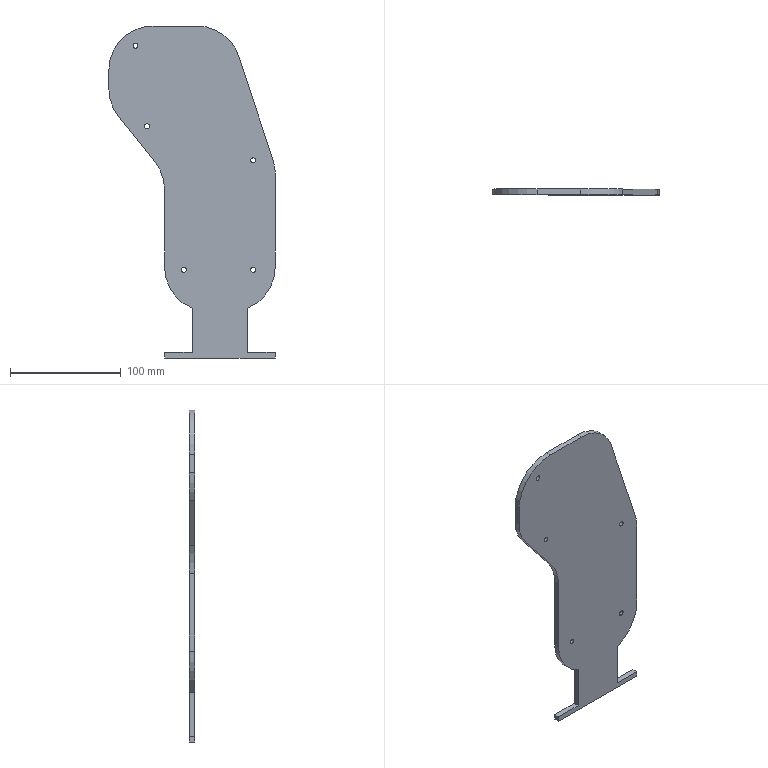Component | SolidWorks | FlatJawHousing-1 | 1 solid | 32 faces | box 150.39 x 5 x 300 mm | volume 146943 mm3 | cylinder 17 | plane 15 | commonest cylinder face diameters 4.5 x10 80 x7
build123d program:
from build123d import *

# Parameters (mm, degrees)
BOSS_EXTRUDE1_DEPTH = 5
SKETCH2_R           = 2.25
CUT_EXTRUDE1_DEPTH  = 10


with BuildPart() as part:
    # Sketch1 → Boss-Extrude1 (new body)
    with BuildSketch(Plane.XY):
        with BuildLine():
            Line((0, 111.584), (0, 95.56))
            Line((0, 95.56), (0, 52.34))
            Line((0, 52.34), (5, 52.34))
            Line((5, 52.34), (5, 77.34))
            Line((5, 77.34), (45, 77.34))
            ThreePointArc((45, 77.34), (59.72, 59.173), (82.081, 52.34))
            Line((82.081, 52.34), (152.399, 52.34))
            ThreePointArc((152.399, 52.34), (165.69, 50.067), (177.471, 43.507))
            Line((177.471, 43.507), (218.149, 10.784))
            ThreePointArc((218.149, 10.784), (229.929, 4.224), (243.221, 1.951))
            Line((243.221, 1.951), (260, 1.951))
            ThreePointArc((260, 1.951), (288.284, 13.667), (300, 41.951))
            Line((300, 41.951), (300, 81.523))
            ThreePointArc((300, 81.523), (292.396, 104.986), (272.474, 119.528))
            Line((272.474, 119.528), (178.577, 150.345))
            ThreePointArc((178.577, 150.345), (172.42, 151.838), (166.104, 152.34))
            Line((166.104, 152.34), (82.081, 152.34))
            ThreePointArc((82.081, 152.34), (59.72, 145.506), (45, 127.34))
            Line((45, 127.34), (5, 127.34))
            Line((5, 127.34), (5, 152.34))
            Line((5, 152.34), (0, 152.34))
            Line((0, 152.34), (0, 111.584))
        make_face()
    extrude(amount=BOSS_EXTRUDE1_DEPTH)

    # Sketch2 → Cut-Extrude1 (cut)
    with BuildSketch(Plane.XY.offset(5)):
        with Locations((79.643, 69.69)):
            Circle(SKETCH2_R)
        with Locations((79.643, 132.549)):
            Circle(SKETCH2_R)
        with Locations((178.581, 132.549)):
            Circle(SKETCH2_R)
        with Locations((209.296, 36.501)):
            Circle(SKETCH2_R)
        with Locations((282.295, 26.112)):
            Circle(SKETCH2_R)
    extrude(amount=-CUT_EXTRUDE1_DEPTH, mode=Mode.SUBTRACT)


solid = part.part

# Placed as in the assembly
solid = solid.moved(Location((361.097, 1552.5, -2182.934), (-90, 0, -90)))
STEP:
#1=COLOUR_RGB('',0.7922,0.8196,0.9333);
#2=FILL_AREA_STYLE_COLOUR('',#1);
#3=FILL_AREA_STYLE('',(#2));
#4=SURFACE_STYLE_FILL_AREA(#3);
#5=SURFACE_SIDE_STYLE('',(#4));
#6=SURFACE_STYLE_USAGE(.BOTH.,#5);
#7=PRESENTATION_STYLE_ASSIGNMENT((#6));
#8=CARTESIAN_POINT('',(15.244,61.122,-74.917));
#9=VERTEX_POINT('',#8);
#10=CARTESIAN_POINT('',(15.244,61.122,-74.74));
#11=VERTEX_POINT('',#10);
#12=CARTESIAN_POINT('',(15.244,61.122,-74.828));
#13=DIRECTION('',(0.,1.,-0.));
#14=DIRECTION('',(0.,0.,1.));
#15=AXIS2_PLACEMENT_3D('',#12,#13,#14);
#16=CIRCLE('',#15,0.08858);
#17=EDGE_CURVE('',#9,#11,#16,.T.);
#18=ORIENTED_EDGE('',*,*,#17,.F.);
#19=CARTESIAN_POINT('',(15.244,61.319,-74.917));
#20=VERTEX_POINT('',#19);
#21=CARTESIAN_POINT('',(15.244,60.925,-74.917));
#22=DIRECTION('',(0.,1.,-0.));
#23=VECTOR('',#22,39.37);
#24=LINE('',#21,#23);
#25=EDGE_CURVE('',#9,#20,#24,.T.);
#26=ORIENTED_EDGE('',*,*,#25,.T.);
#27=CARTESIAN_POINT('',(15.244,61.319,-74.74));
#28=VERTEX_POINT('',#27);
#29=CARTESIAN_POINT('',(15.244,61.319,-74.828));
#30=DIRECTION('',(0.,1.,-0.));
#31=DIRECTION('',(0.,0.,1.));
#32=AXIS2_PLACEMENT_3D('',#29,#30,#31);
#33=CIRCLE('',#32,0.08858);
#34=EDGE_CURVE('',#20,#28,#33,.T.);
#35=ORIENTED_EDGE('',*,*,#34,.T.);
#36=CARTESIAN_POINT('',(15.244,60.925,-74.74));
#37=DIRECTION('',(0.,1.,-0.));
#38=VECTOR('',#37,39.37);
#39=LINE('',#36,#38);
#40=EDGE_CURVE('',#11,#28,#39,.T.);
#41=ORIENTED_EDGE('',*,*,#40,.F.);
#42=EDGE_LOOP('',(#18,#26,#35,#41));
#43=FACE_OUTER_BOUND('',#42,.T.);
#44=CARTESIAN_POINT('',(15.244,60.925,-74.828));
#45=DIRECTION('',(0.,1.,-0.));
#46=DIRECTION('',(0.,0.,1.));
#47=AXIS2_PLACEMENT_3D('',#44,#45,#46);
#48=CYLINDRICAL_SURFACE('',#47,0.08858);
#49=ADVANCED_FACE('',(#43),#48,.F.);
#50=CARTESIAN_POINT('',(15.653,61.122,-77.791));
#51=VERTEX_POINT('',#50);
#52=CARTESIAN_POINT('',(15.653,61.122,-77.614));
#53=VERTEX_POINT('',#52);
#54=CARTESIAN_POINT('',(15.653,61.122,-77.702));
#55=DIRECTION('',(0.,1.,-0.));
#56=DIRECTION('',(0.,0.,1.));
#57=AXIS2_PLACEMENT_3D('',#54,#55,#56);
#58=CIRCLE('',#57,0.08858);
#59=EDGE_CURVE('',#51,#53,#58,.T.);
#60=ORIENTED_EDGE('',*,*,#59,.F.);
#61=CARTESIAN_POINT('',(15.653,61.319,-77.791));
#62=VERTEX_POINT('',#61);
#63=CARTESIAN_POINT('',(15.653,60.925,-77.791));
#64=DIRECTION('',(0.,1.,-0.));
#65=VECTOR('',#64,39.37);
#66=LINE('',#63,#65);
#67=EDGE_CURVE('',#51,#62,#66,.T.);
#68=ORIENTED_EDGE('',*,*,#67,.T.);
#69=CARTESIAN_POINT('',(15.653,61.319,-77.614));
#70=VERTEX_POINT('',#69);
#71=CARTESIAN_POINT('',(15.653,61.319,-77.702));
#72=DIRECTION('',(0.,1.,-0.));
#73=DIRECTION('',(0.,0.,1.));
#74=AXIS2_PLACEMENT_3D('',#71,#72,#73);
#75=CIRCLE('',#74,0.08858);
#76=EDGE_CURVE('',#62,#70,#75,.T.);
#77=ORIENTED_EDGE('',*,*,#76,.T.);
#78=CARTESIAN_POINT('',(15.653,60.925,-77.614));
#79=DIRECTION('',(0.,1.,-0.));
#80=VECTOR('',#79,39.37);
#81=LINE('',#78,#80);
#82=EDGE_CURVE('',#53,#70,#81,.T.);
#83=ORIENTED_EDGE('',*,*,#82,.F.);
#84=EDGE_LOOP('',(#60,#68,#77,#83));
#85=FACE_OUTER_BOUND('',#84,.T.);
#86=CARTESIAN_POINT('',(15.653,60.925,-77.702));
#87=DIRECTION('',(0.,1.,-0.));
#88=DIRECTION('',(0.,0.,1.));
#89=AXIS2_PLACEMENT_3D('',#86,#87,#88);
#90=CYLINDRICAL_SURFACE('',#89,0.08858);
#91=ADVANCED_FACE('',(#85),#90,.F.);
#92=CARTESIAN_POINT('',(19.435,61.122,-79.));
#93=VERTEX_POINT('',#92);
#94=CARTESIAN_POINT('',(19.435,61.122,-78.823));
#95=VERTEX_POINT('',#94);
#96=CARTESIAN_POINT('',(19.435,61.122,-78.912));
#97=DIRECTION('',(0.,1.,-0.));
#98=DIRECTION('',(0.,0.,1.));
#99=AXIS2_PLACEMENT_3D('',#96,#97,#98);
#100=CIRCLE('',#99,0.08858);
#101=EDGE_CURVE('',#93,#95,#100,.T.);
#102=ORIENTED_EDGE('',*,*,#101,.F.);
#103=CARTESIAN_POINT('',(19.435,61.319,-79.));
#104=VERTEX_POINT('',#103);
#105=CARTESIAN_POINT('',(19.435,60.925,-79.));
#106=DIRECTION('',(0.,1.,-0.));
#107=VECTOR('',#106,39.37);
#108=LINE('',#105,#107);
#109=EDGE_CURVE('',#93,#104,#108,.T.);
#110=ORIENTED_EDGE('',*,*,#109,.T.);
#111=CARTESIAN_POINT('',(19.435,61.319,-78.823));
#112=VERTEX_POINT('',#111);
#113=CARTESIAN_POINT('',(19.435,61.319,-78.912));
#114=DIRECTION('',(0.,1.,-0.));
#115=DIRECTION('',(0.,0.,1.));
#116=AXIS2_PLACEMENT_3D('',#113,#114,#115);
#117=CIRCLE('',#116,0.08858);
#118=EDGE_CURVE('',#104,#112,#117,.T.);
#119=ORIENTED_EDGE('',*,*,#118,.T.);
#120=CARTESIAN_POINT('',(19.435,60.925,-78.823));
#121=DIRECTION('',(0.,1.,-0.));
#122=VECTOR('',#121,39.37);
#123=LINE('',#120,#122);
#124=EDGE_CURVE('',#95,#112,#123,.T.);
#125=ORIENTED_EDGE('',*,*,#124,.F.);
#126=EDGE_LOOP('',(#102,#110,#119,#125));
#127=FACE_OUTER_BOUND('',#126,.T.);
#128=CARTESIAN_POINT('',(19.435,60.925,-78.912));
#129=DIRECTION('',(0.,1.,-0.));
#130=DIRECTION('',(0.,0.,1.));
#131=AXIS2_PLACEMENT_3D('',#128,#129,#130);
#132=CYLINDRICAL_SURFACE('',#131,0.08858);
#133=ADVANCED_FACE('',(#127),#132,.F.);
#134=CARTESIAN_POINT('',(19.435,61.122,-82.895));
#135=VERTEX_POINT('',#134);
#136=CARTESIAN_POINT('',(19.435,61.122,-82.718));
#137=VERTEX_POINT('',#136);
#138=CARTESIAN_POINT('',(19.435,61.122,-82.807));
#139=DIRECTION('',(0.,1.,-0.));
#140=DIRECTION('',(0.,0.,1.));
#141=AXIS2_PLACEMENT_3D('',#138,#139,#140);
#142=CIRCLE('',#141,0.08858);
#143=EDGE_CURVE('',#135,#137,#142,.T.);
#144=ORIENTED_EDGE('',*,*,#143,.F.);
#145=CARTESIAN_POINT('',(19.435,61.319,-82.895));
#146=VERTEX_POINT('',#145);
#147=CARTESIAN_POINT('',(19.435,60.925,-82.895));
#148=DIRECTION('',(0.,1.,-0.));
#149=VECTOR('',#148,39.37);
#150=LINE('',#147,#149);
#151=EDGE_CURVE('',#135,#146,#150,.T.);
#152=ORIENTED_EDGE('',*,*,#151,.T.);
#153=CARTESIAN_POINT('',(19.435,61.319,-82.718));
#154=VERTEX_POINT('',#153);
#155=CARTESIAN_POINT('',(19.435,61.319,-82.807));
#156=DIRECTION('',(0.,1.,-0.));
#157=DIRECTION('',(0.,0.,1.));
#158=AXIS2_PLACEMENT_3D('',#155,#156,#157);
#159=CIRCLE('',#158,0.08858);
#160=EDGE_CURVE('',#146,#154,#159,.T.);
#161=ORIENTED_EDGE('',*,*,#160,.T.);
#162=CARTESIAN_POINT('',(19.435,60.925,-82.718));
#163=DIRECTION('',(0.,1.,-0.));
#164=VECTOR('',#163,39.37);
#165=LINE('',#162,#164);
#166=EDGE_CURVE('',#137,#154,#165,.T.);
#167=ORIENTED_EDGE('',*,*,#166,.F.);
#168=EDGE_LOOP('',(#144,#152,#161,#167));
#169=FACE_OUTER_BOUND('',#168,.T.);
#170=CARTESIAN_POINT('',(19.435,60.925,-82.807));
#171=DIRECTION('',(0.,1.,-0.));
#172=DIRECTION('',(0.,0.,1.));
#173=AXIS2_PLACEMENT_3D('',#170,#171,#172);
#174=CYLINDRICAL_SURFACE('',#173,0.08858);
#175=ADVANCED_FACE('',(#169),#174,.F.);
#176=CARTESIAN_POINT('',(16.96,61.122,-82.895));
#177=VERTEX_POINT('',#176);
#178=CARTESIAN_POINT('',(16.96,61.122,-82.718));
#179=VERTEX_POINT('',#178);
#180=CARTESIAN_POINT('',(16.96,61.122,-82.807));
#181=DIRECTION('',(0.,1.,-0.));
#182=DIRECTION('',(0.,0.,1.));
#183=AXIS2_PLACEMENT_3D('',#180,#181,#182);
#184=CIRCLE('',#183,0.08858);
#185=EDGE_CURVE('',#177,#179,#184,.T.);
#186=ORIENTED_EDGE('',*,*,#185,.F.);
#187=CARTESIAN_POINT('',(16.96,61.319,-82.895));
#188=VERTEX_POINT('',#187);
#189=CARTESIAN_POINT('',(16.96,60.925,-82.895));
#190=DIRECTION('',(0.,1.,-0.));
#191=VECTOR('',#190,39.37);
#192=LINE('',#189,#191);
#193=EDGE_CURVE('',#177,#188,#192,.T.);
#194=ORIENTED_EDGE('',*,*,#193,.T.);
#195=CARTESIAN_POINT('',(16.96,61.319,-82.718));
#196=VERTEX_POINT('',#195);
#197=CARTESIAN_POINT('',(16.96,61.319,-82.807));
#198=DIRECTION('',(0.,1.,-0.));
#199=DIRECTION('',(0.,0.,1.));
#200=AXIS2_PLACEMENT_3D('',#197,#198,#199);
#201=CIRCLE('',#200,0.08858);
#202=EDGE_CURVE('',#188,#196,#201,.T.);
#203=ORIENTED_EDGE('',*,*,#202,.T.);
#204=CARTESIAN_POINT('',(16.96,60.925,-82.718));
#205=DIRECTION('',(0.,1.,-0.));
#206=VECTOR('',#205,39.37);
#207=LINE('',#204,#206);
#208=EDGE_CURVE('',#179,#196,#207,.T.);
#209=ORIENTED_EDGE('',*,*,#208,.F.);
#210=EDGE_LOOP('',(#186,#194,#203,#209));
#211=FACE_OUTER_BOUND('',#210,.T.);
#212=CARTESIAN_POINT('',(16.96,60.925,-82.807));
#213=DIRECTION('',(0.,1.,-0.));
#214=DIRECTION('',(0.,0.,1.));
#215=AXIS2_PLACEMENT_3D('',#212,#213,#214);
#216=CYLINDRICAL_SURFACE('',#215,0.08858);
#217=ADVANCED_FACE('',(#211),#216,.F.);
#218=CARTESIAN_POINT('',(20.136,61.122,-78.912));
#219=VERTEX_POINT('',#218);
#220=CARTESIAN_POINT('',(20.214,61.122,-79.403));
#221=VERTEX_POINT('',#220);
#222=CARTESIAN_POINT('',(18.639,61.122,-79.403));
#223=DIRECTION('',(0.,1.,-0.));
#224=DIRECTION('',(0.,0.,1.));
#225=AXIS2_PLACEMENT_3D('',#222,#223,#224);
#226=CIRCLE('',#225,1.575);
#227=EDGE_CURVE('',#219,#221,#226,.T.);
#228=ORIENTED_EDGE('',*,*,#227,.T.);
#229=CARTESIAN_POINT('',(20.214,61.319,-79.403));
#230=VERTEX_POINT('',#229);
#231=CARTESIAN_POINT('',(20.214,61.319,-79.403));
#232=DIRECTION('',(0.,-1.,0.));
#233=VECTOR('',#232,39.37);
#234=LINE('',#231,#233);
#235=EDGE_CURVE('',#230,#221,#234,.T.);
#236=ORIENTED_EDGE('',*,*,#235,.F.);
#237=CARTESIAN_POINT('',(20.136,61.319,-78.912));
#238=VERTEX_POINT('',#237);
#239=CARTESIAN_POINT('',(18.639,61.319,-79.403));
#240=DIRECTION('',(0.,1.,-0.));
#241=DIRECTION('',(0.,0.,1.));
#242=AXIS2_PLACEMENT_3D('',#239,#240,#241);
#243=CIRCLE('',#242,1.575);
#244=EDGE_CURVE('',#238,#230,#243,.T.);
#245=ORIENTED_EDGE('',*,*,#244,.F.);
#246=CARTESIAN_POINT('',(20.136,61.319,-78.912));
#247=DIRECTION('',(0.,-1.,0.));
#248=VECTOR('',#247,39.37);
#249=LINE('',#246,#248);
#250=EDGE_CURVE('',#238,#219,#249,.T.);
#251=ORIENTED_EDGE('',*,*,#250,.T.);
#252=EDGE_LOOP('',(#228,#236,#245,#251));
#253=FACE_OUTER_BOUND('',#252,.T.);
#254=CARTESIAN_POINT('',(18.639,61.319,-79.403));
#255=DIRECTION('',(0.,-1.,0.));
#256=DIRECTION('',(0.,0.,-1.));
#257=AXIS2_PLACEMENT_3D('',#254,#255,#256);
#258=CYLINDRICAL_SURFACE('',#257,1.575);
#259=ADVANCED_FACE('',(#253),#258,.T.);
#260=CARTESIAN_POINT('',(20.214,61.122,-82.711));
#261=VERTEX_POINT('',#260);
#262=CARTESIAN_POINT('',(20.214,61.122,-79.403));
#263=DIRECTION('',(0.,-0.,-1.));
#264=VECTOR('',#263,39.37);
#265=LINE('',#262,#264);
#266=EDGE_CURVE('',#221,#261,#265,.T.);
#267=ORIENTED_EDGE('',*,*,#266,.T.);
#268=CARTESIAN_POINT('',(20.214,61.319,-82.711));
#269=VERTEX_POINT('',#268);
#270=CARTESIAN_POINT('',(20.214,61.319,-82.711));
#271=DIRECTION('',(0.,-1.,0.));
#272=VECTOR('',#271,39.37);
#273=LINE('',#270,#272);
#274=EDGE_CURVE('',#269,#261,#273,.T.);
#275=ORIENTED_EDGE('',*,*,#274,.F.);
#276=CARTESIAN_POINT('',(20.214,61.319,-79.403));
#277=DIRECTION('',(0.,-0.,-1.));
#278=VECTOR('',#277,39.37);
#279=LINE('',#276,#278);
#280=EDGE_CURVE('',#230,#269,#279,.T.);
#281=ORIENTED_EDGE('',*,*,#280,.F.);
#282=ORIENTED_EDGE('',*,*,#235,.T.);
#283=EDGE_LOOP('',(#267,#275,#281,#282));
#284=FACE_OUTER_BOUND('',#283,.T.);
#285=CARTESIAN_POINT('',(20.214,61.319,-79.403));
#286=DIRECTION('',(-1.,-0.,-0.));
#287=DIRECTION('',(-0.,0.,1.));
#288=AXIS2_PLACEMENT_3D('',#285,#286,#287);
#289=PLANE('',#288);
#290=ADVANCED_FACE('',(#284),#289,.F.);
#291=CARTESIAN_POINT('',(19.23,61.122,-84.171));
#292=VERTEX_POINT('',#291);
#293=CARTESIAN_POINT('',(18.639,61.122,-82.711));
#294=DIRECTION('',(0.,1.,-0.));
#295=DIRECTION('',(0.,0.,1.));
#296=AXIS2_PLACEMENT_3D('',#293,#294,#295);
#297=CIRCLE('',#296,1.575);
#298=EDGE_CURVE('',#261,#292,#297,.T.);
#299=ORIENTED_EDGE('',*,*,#298,.T.);
#300=CARTESIAN_POINT('',(19.23,61.319,-84.171));
#301=VERTEX_POINT('',#300);
#302=CARTESIAN_POINT('',(19.23,61.319,-84.171));
#303=DIRECTION('',(0.,-1.,0.));
#304=VECTOR('',#303,39.37);
#305=LINE('',#302,#304);
#306=EDGE_CURVE('',#301,#292,#305,.T.);
#307=ORIENTED_EDGE('',*,*,#306,.F.);
#308=CARTESIAN_POINT('',(18.639,61.319,-82.711));
#309=DIRECTION('',(0.,1.,-0.));
#310=DIRECTION('',(0.,0.,1.));
#311=AXIS2_PLACEMENT_3D('',#308,#309,#310);
#312=CIRCLE('',#311,1.575);
#313=EDGE_CURVE('',#269,#301,#312,.T.);
#314=ORIENTED_EDGE('',*,*,#313,.F.);
#315=ORIENTED_EDGE('',*,*,#274,.T.);
#316=EDGE_LOOP('',(#299,#307,#314,#315));
#317=FACE_OUTER_BOUND('',#316,.T.);
#318=CARTESIAN_POINT('',(18.639,61.319,-82.711));
#319=DIRECTION('',(0.,-1.,0.));
#320=DIRECTION('',(0.,0.,-1.));
#321=AXIS2_PLACEMENT_3D('',#318,#319,#320);
#322=CYLINDRICAL_SURFACE('',#321,1.575);
#323=ADVANCED_FACE('',(#317),#322,.T.);
#324=CARTESIAN_POINT('',(19.23,61.122,-85.745));
#325=VERTEX_POINT('',#324);
#326=CARTESIAN_POINT('',(19.23,61.122,-84.171));
#327=DIRECTION('',(0.,-0.,-1.));
#328=VECTOR('',#327,39.37);
#329=LINE('',#326,#328);
#330=EDGE_CURVE('',#292,#325,#329,.T.);
#331=ORIENTED_EDGE('',*,*,#330,.T.);
#332=CARTESIAN_POINT('',(19.23,61.319,-85.745));
#333=VERTEX_POINT('',#332);
#334=CARTESIAN_POINT('',(19.23,61.319,-85.745));
#335=DIRECTION('',(0.,-1.,0.));
#336=VECTOR('',#335,39.37);
#337=LINE('',#334,#336);
#338=EDGE_CURVE('',#333,#325,#337,.T.);
#339=ORIENTED_EDGE('',*,*,#338,.F.);
#340=CARTESIAN_POINT('',(19.23,61.319,-84.171));
#341=DIRECTION('',(0.,-0.,-1.));
#342=VECTOR('',#341,39.37);
#343=LINE('',#340,#342);
#344=EDGE_CURVE('',#301,#333,#343,.T.);
#345=ORIENTED_EDGE('',*,*,#344,.F.);
#346=ORIENTED_EDGE('',*,*,#306,.T.);
#347=EDGE_LOOP('',(#331,#339,#345,#346));
#348=FACE_OUTER_BOUND('',#347,.T.);
#349=CARTESIAN_POINT('',(19.23,61.319,-84.171));
#350=DIRECTION('',(-1.,0.,0.));
#351=DIRECTION('',(0.,-1.,0.));
#352=AXIS2_PLACEMENT_3D('',#349,#350,#351);
#353=PLANE('',#352);
#354=ADVANCED_FACE('',(#348),#353,.F.);
#355=CARTESIAN_POINT('',(20.214,61.122,-85.745));
#356=VERTEX_POINT('',#355);
#357=CARTESIAN_POINT('',(19.23,61.122,-85.745));
#358=DIRECTION('',(1.,0.,0.));
#359=VECTOR('',#358,39.37);
#360=LINE('',#357,#359);
#361=EDGE_CURVE('',#325,#356,#360,.T.);
#362=ORIENTED_EDGE('',*,*,#361,.T.);
#363=CARTESIAN_POINT('',(20.214,61.319,-85.745));
#364=VERTEX_POINT('',#363);
#365=CARTESIAN_POINT('',(20.214,61.319,-85.745));
#366=DIRECTION('',(0.,-1.,0.));
#367=VECTOR('',#366,39.37);
#368=LINE('',#365,#367);
#369=EDGE_CURVE('',#364,#356,#368,.T.);
#370=ORIENTED_EDGE('',*,*,#369,.F.);
#371=CARTESIAN_POINT('',(19.23,61.319,-85.745));
#372=DIRECTION('',(1.,0.,0.));
#373=VECTOR('',#372,39.37);
#374=LINE('',#371,#373);
#375=EDGE_CURVE('',#333,#364,#374,.T.);
#376=ORIENTED_EDGE('',*,*,#375,.F.);
#377=ORIENTED_EDGE('',*,*,#338,.T.);
#378=EDGE_LOOP('',(#362,#370,#376,#377));
#379=FACE_OUTER_BOUND('',#378,.T.);
#380=CARTESIAN_POINT('',(19.23,61.319,-85.745));
#381=DIRECTION('',(0.,-0.,-1.));
#382=DIRECTION('',(0.,1.,-0.));
#383=AXIS2_PLACEMENT_3D('',#380,#381,#382);
#384=PLANE('',#383);
#385=ADVANCED_FACE('',(#379),#384,.F.);
#386=CARTESIAN_POINT('',(20.214,61.122,-85.942));
#387=VERTEX_POINT('',#386);
#388=CARTESIAN_POINT('',(20.214,61.122,-85.745));
#389=DIRECTION('',(0.,-0.,-1.));
#390=VECTOR('',#389,39.37);
#391=LINE('',#388,#390);
#392=EDGE_CURVE('',#356,#387,#391,.T.);
#393=ORIENTED_EDGE('',*,*,#392,.T.);
#394=CARTESIAN_POINT('',(20.214,61.319,-85.942));
#395=VERTEX_POINT('',#394);
#396=CARTESIAN_POINT('',(20.214,61.319,-85.942));
#397=DIRECTION('',(0.,-1.,0.));
#398=VECTOR('',#397,39.37);
#399=LINE('',#396,#398);
#400=EDGE_CURVE('',#395,#387,#399,.T.);
#401=ORIENTED_EDGE('',*,*,#400,.F.);
#402=CARTESIAN_POINT('',(20.214,61.319,-85.745));
#403=DIRECTION('',(0.,-0.,-1.));
#404=VECTOR('',#403,39.37);
#405=LINE('',#402,#404);
#406=EDGE_CURVE('',#364,#395,#405,.T.);
#407=ORIENTED_EDGE('',*,*,#406,.F.);
#408=ORIENTED_EDGE('',*,*,#369,.T.);
#409=EDGE_LOOP('',(#393,#401,#407,#408));
#410=FACE_OUTER_BOUND('',#409,.T.);
#411=CARTESIAN_POINT('',(20.214,61.319,-85.745));
#412=DIRECTION('',(-1.,0.,0.));
#413=DIRECTION('',(0.,-1.,0.));
#414=AXIS2_PLACEMENT_3D('',#411,#412,#413);
#415=PLANE('',#414);
#416=ADVANCED_FACE('',(#410),#415,.F.);
#417=CARTESIAN_POINT('',(16.277,61.122,-85.942));
#418=VERTEX_POINT('',#417);
#419=CARTESIAN_POINT('',(17.979,61.122,-85.942));
#420=DIRECTION('',(-1.,0.,0.));
#421=VECTOR('',#420,39.37);
#422=LINE('',#419,#421);
#423=EDGE_CURVE('',#387,#418,#422,.T.);
#424=ORIENTED_EDGE('',*,*,#423,.T.);
#425=CARTESIAN_POINT('',(16.277,61.319,-85.942));
#426=VERTEX_POINT('',#425);
#427=CARTESIAN_POINT('',(16.277,61.319,-85.942));
#428=DIRECTION('',(0.,-1.,0.));
#429=VECTOR('',#428,39.37);
#430=LINE('',#427,#429);
#431=EDGE_CURVE('',#426,#418,#430,.T.);
#432=ORIENTED_EDGE('',*,*,#431,.F.);
#433=CARTESIAN_POINT('',(20.214,61.319,-85.942));
#434=DIRECTION('',(-1.,0.,0.));
#435=VECTOR('',#434,39.37);
#436=LINE('',#433,#435);
#437=EDGE_CURVE('',#395,#426,#436,.T.);
#438=ORIENTED_EDGE('',*,*,#437,.F.);
#439=ORIENTED_EDGE('',*,*,#400,.T.);
#440=EDGE_LOOP('',(#424,#432,#438,#439));
#441=FACE_OUTER_BOUND('',#440,.T.);
#442=CARTESIAN_POINT('',(17.979,61.319,-85.942));
#443=DIRECTION('',(0.,0.,1.));
#444=DIRECTION('',(0.,-1.,0.));
#445=AXIS2_PLACEMENT_3D('',#442,#443,#444);
#446=PLANE('',#445);
#447=ADVANCED_FACE('',(#441),#446,.F.);
#448=CARTESIAN_POINT('',(16.277,61.122,-85.745));
#449=VERTEX_POINT('',#448);
#450=CARTESIAN_POINT('',(16.277,61.122,-85.942));
#451=DIRECTION('',(0.,0.,1.));
#452=VECTOR('',#451,39.37);
#453=LINE('',#450,#452);
#454=EDGE_CURVE('',#418,#449,#453,.T.);
#455=ORIENTED_EDGE('',*,*,#454,.T.);
#456=CARTESIAN_POINT('',(16.277,61.319,-85.745));
#457=VERTEX_POINT('',#456);
#458=CARTESIAN_POINT('',(16.277,61.319,-85.745));
#459=DIRECTION('',(0.,-1.,0.));
#460=VECTOR('',#459,39.37);
#461=LINE('',#458,#460);
#462=EDGE_CURVE('',#457,#449,#461,.T.);
#463=ORIENTED_EDGE('',*,*,#462,.F.);
#464=CARTESIAN_POINT('',(16.277,61.319,-85.942));
#465=DIRECTION('',(0.,0.,1.));
#466=VECTOR('',#465,39.37);
#467=LINE('',#464,#466);
#468=EDGE_CURVE('',#426,#457,#467,.T.);
#469=ORIENTED_EDGE('',*,*,#468,.F.);
#470=ORIENTED_EDGE('',*,*,#431,.T.);
#471=EDGE_LOOP('',(#455,#463,#469,#470));
#472=FACE_OUTER_BOUND('',#471,.T.);
#473=CARTESIAN_POINT('',(16.277,61.319,-85.942));
#474=DIRECTION('',(1.,0.,0.));
#475=DIRECTION('',(0.,1.,-0.));
#476=AXIS2_PLACEMENT_3D('',#473,#474,#475);
#477=PLANE('',#476);
#478=ADVANCED_FACE('',(#472),#477,.F.);
#479=CARTESIAN_POINT('',(17.261,61.122,-85.745));
#480=VERTEX_POINT('',#479);
#481=CARTESIAN_POINT('',(16.277,61.122,-85.745));
#482=DIRECTION('',(1.,0.,0.));
#483=VECTOR('',#482,39.37);
#484=LINE('',#481,#483);
#485=EDGE_CURVE('',#449,#480,#484,.T.);
#486=ORIENTED_EDGE('',*,*,#485,.T.);
#487=CARTESIAN_POINT('',(17.261,61.319,-85.745));
#488=VERTEX_POINT('',#487);
#489=CARTESIAN_POINT('',(17.261,61.319,-85.745));
#490=DIRECTION('',(0.,-1.,0.));
#491=VECTOR('',#490,39.37);
#492=LINE('',#489,#491);
#493=EDGE_CURVE('',#488,#480,#492,.T.);
#494=ORIENTED_EDGE('',*,*,#493,.F.);
#495=CARTESIAN_POINT('',(16.277,61.319,-85.745));
#496=DIRECTION('',(1.,0.,0.));
#497=VECTOR('',#496,39.37);
#498=LINE('',#495,#497);
#499=EDGE_CURVE('',#457,#488,#498,.T.);
#500=ORIENTED_EDGE('',*,*,#499,.F.);
#501=ORIENTED_EDGE('',*,*,#462,.T.);
#502=EDGE_LOOP('',(#486,#494,#500,#501));
#503=FACE_OUTER_BOUND('',#502,.T.);
#504=CARTESIAN_POINT('',(16.277,61.319,-85.745));
#505=DIRECTION('',(0.,-0.,-1.));
#506=DIRECTION('',(0.,1.,-0.));
#507=AXIS2_PLACEMENT_3D('',#504,#505,#506);
#508=PLANE('',#507);
#509=ADVANCED_FACE('',(#503),#508,.F.);
#510=CARTESIAN_POINT('',(17.261,61.122,-84.171));
#511=VERTEX_POINT('',#510);
#512=CARTESIAN_POINT('',(17.261,61.122,-85.745));
#513=DIRECTION('',(0.,0.,1.));
#514=VECTOR('',#513,39.37);
#515=LINE('',#512,#514);
#516=EDGE_CURVE('',#480,#511,#515,.T.);
#517=ORIENTED_EDGE('',*,*,#516,.T.);
#518=CARTESIAN_POINT('',(17.261,61.319,-84.171));
#519=VERTEX_POINT('',#518);
#520=CARTESIAN_POINT('',(17.261,61.319,-84.171));
#521=DIRECTION('',(0.,-1.,0.));
#522=VECTOR('',#521,39.37);
#523=LINE('',#520,#522);
#524=EDGE_CURVE('',#519,#511,#523,.T.);
#525=ORIENTED_EDGE('',*,*,#524,.F.);
#526=CARTESIAN_POINT('',(17.261,61.319,-85.745));
#527=DIRECTION('',(0.,0.,1.));
#528=VECTOR('',#527,39.37);
#529=LINE('',#526,#528);
#530=EDGE_CURVE('',#488,#519,#529,.T.);
#531=ORIENTED_EDGE('',*,*,#530,.F.);
#532=ORIENTED_EDGE('',*,*,#493,.T.);
#533=EDGE_LOOP('',(#517,#525,#531,#532));
#534=FACE_OUTER_BOUND('',#533,.T.);
#535=CARTESIAN_POINT('',(17.261,61.319,-85.745));
#536=DIRECTION('',(1.,0.,0.));
#537=DIRECTION('',(0.,1.,-0.));
#538=AXIS2_PLACEMENT_3D('',#535,#536,#537);
#539=PLANE('',#538);
#540=ADVANCED_FACE('',(#534),#539,.F.);
#541=CARTESIAN_POINT('',(16.277,61.122,-82.711));
#542=VERTEX_POINT('',#541);
#543=CARTESIAN_POINT('',(17.852,61.122,-82.711));
#544=DIRECTION('',(0.,1.,-0.));
#545=DIRECTION('',(0.,0.,1.));
#546=AXIS2_PLACEMENT_3D('',#543,#544,#545);
#547=CIRCLE('',#546,1.575);
#548=EDGE_CURVE('',#511,#542,#547,.T.);
#549=ORIENTED_EDGE('',*,*,#548,.T.);
#550=CARTESIAN_POINT('',(16.277,61.319,-82.711));
#551=VERTEX_POINT('',#550);
#552=CARTESIAN_POINT('',(16.277,61.319,-82.711));
#553=DIRECTION('',(0.,-1.,0.));
#554=VECTOR('',#553,39.37);
#555=LINE('',#552,#554);
#556=EDGE_CURVE('',#551,#542,#555,.T.);
#557=ORIENTED_EDGE('',*,*,#556,.F.);
#558=CARTESIAN_POINT('',(17.852,61.319,-82.711));
#559=DIRECTION('',(0.,1.,-0.));
#560=DIRECTION('',(0.,0.,1.));
#561=AXIS2_PLACEMENT_3D('',#558,#559,#560);
#562=CIRCLE('',#561,1.575);
#563=EDGE_CURVE('',#519,#551,#562,.T.);
#564=ORIENTED_EDGE('',*,*,#563,.F.);
#565=ORIENTED_EDGE('',*,*,#524,.T.);
#566=EDGE_LOOP('',(#549,#557,#564,#565));
#567=FACE_OUTER_BOUND('',#566,.T.);
#568=CARTESIAN_POINT('',(17.852,61.319,-82.711));
#569=DIRECTION('',(0.,-1.,0.));
#570=DIRECTION('',(0.,0.,-1.));
#571=AXIS2_PLACEMENT_3D('',#568,#569,#570);
#572=CYLINDRICAL_SURFACE('',#571,1.575);
#573=ADVANCED_FACE('',(#567),#572,.T.);
#574=CARTESIAN_POINT('',(16.277,61.122,-79.942));
#575=VERTEX_POINT('',#574);
#576=CARTESIAN_POINT('',(16.277,61.122,-82.711));
#577=DIRECTION('',(-0.,0.,1.));
#578=VECTOR('',#577,39.37);
#579=LINE('',#576,#578);
#580=EDGE_CURVE('',#542,#575,#579,.T.);
#581=ORIENTED_EDGE('',*,*,#580,.T.);
#582=CARTESIAN_POINT('',(16.277,61.319,-79.942));
#583=VERTEX_POINT('',#582);
#584=CARTESIAN_POINT('',(16.277,61.319,-79.942));
#585=DIRECTION('',(0.,-1.,0.));
#586=VECTOR('',#585,39.37);
#587=LINE('',#584,#586);
#588=EDGE_CURVE('',#583,#575,#587,.T.);
#589=ORIENTED_EDGE('',*,*,#588,.F.);
#590=CARTESIAN_POINT('',(16.277,61.319,-82.711));
#591=DIRECTION('',(-0.,0.,1.));
#592=VECTOR('',#591,39.37);
#593=LINE('',#590,#592);
#594=EDGE_CURVE('',#551,#583,#593,.T.);
#595=ORIENTED_EDGE('',*,*,#594,.F.);
#596=ORIENTED_EDGE('',*,*,#556,.T.);
#597=EDGE_LOOP('',(#581,#589,#595,#596));
#598=FACE_OUTER_BOUND('',#597,.T.);
#599=CARTESIAN_POINT('',(16.277,61.319,-82.711));
#600=DIRECTION('',(1.,0.,0.));
#601=DIRECTION('',(0.,-0.,-1.));
#602=AXIS2_PLACEMENT_3D('',#599,#600,#601);
#603=PLANE('',#602);
#604=ADVANCED_FACE('',(#598),#603,.F.);
#605=CARTESIAN_POINT('',(15.929,61.122,-78.955));
#606=VERTEX_POINT('',#605);
#607=CARTESIAN_POINT('',(14.702,61.122,-79.942));
#608=DIRECTION('',(0.,-1.,0.));
#609=DIRECTION('',(0.,0.,1.));
#610=AXIS2_PLACEMENT_3D('',#607,#608,#609);
#611=CIRCLE('',#610,1.575);
#612=EDGE_CURVE('',#575,#606,#611,.T.);
#613=ORIENTED_EDGE('',*,*,#612,.T.);
#614=CARTESIAN_POINT('',(15.929,61.319,-78.955));
#615=VERTEX_POINT('',#614);
#616=CARTESIAN_POINT('',(15.929,61.319,-78.955));
#617=DIRECTION('',(0.,-1.,0.));
#618=VECTOR('',#617,39.37);
#619=LINE('',#616,#618);
#620=EDGE_CURVE('',#615,#606,#619,.T.);
#621=ORIENTED_EDGE('',*,*,#620,.F.);
#622=CARTESIAN_POINT('',(14.702,61.319,-79.942));
#623=DIRECTION('',(0.,-1.,0.));
#624=DIRECTION('',(0.,0.,1.));
#625=AXIS2_PLACEMENT_3D('',#622,#623,#624);
#626=CIRCLE('',#625,1.575);
#627=EDGE_CURVE('',#583,#615,#626,.T.);
#628=ORIENTED_EDGE('',*,*,#627,.F.);
#629=ORIENTED_EDGE('',*,*,#588,.T.);
#630=EDGE_LOOP('',(#613,#621,#628,#629));
#631=FACE_OUTER_BOUND('',#630,.T.);
#632=CARTESIAN_POINT('',(14.702,61.319,-79.942));
#633=DIRECTION('',(0.,-1.,0.));
#634=DIRECTION('',(0.,0.,-1.));
#635=AXIS2_PLACEMENT_3D('',#632,#633,#634);
#636=CYLINDRICAL_SURFACE('',#635,1.575);
#637=ADVANCED_FACE('',(#631),#636,.F.);
#638=CARTESIAN_POINT('',(14.641,61.122,-77.354));
#639=VERTEX_POINT('',#638);
#640=CARTESIAN_POINT('',(15.929,61.122,-78.955));
#641=DIRECTION('',(-0.6268,0.,0.7792));
#642=VECTOR('',#641,39.37);
#643=LINE('',#640,#642);
#644=EDGE_CURVE('',#606,#639,#643,.T.);
#645=ORIENTED_EDGE('',*,*,#644,.T.);
#646=CARTESIAN_POINT('',(14.641,61.319,-77.354));
#647=VERTEX_POINT('',#646);
#648=CARTESIAN_POINT('',(14.641,61.319,-77.354));
#649=DIRECTION('',(0.,-1.,0.));
#650=VECTOR('',#649,39.37);
#651=LINE('',#648,#650);
#652=EDGE_CURVE('',#647,#639,#651,.T.);
#653=ORIENTED_EDGE('',*,*,#652,.F.);
#654=CARTESIAN_POINT('',(15.929,61.319,-78.955));
#655=DIRECTION('',(-0.6268,0.,0.7792));
#656=VECTOR('',#655,39.37);
#657=LINE('',#654,#656);
#658=EDGE_CURVE('',#615,#647,#657,.T.);
#659=ORIENTED_EDGE('',*,*,#658,.F.);
#660=ORIENTED_EDGE('',*,*,#620,.T.);
#661=EDGE_LOOP('',(#645,#653,#659,#660));
#662=FACE_OUTER_BOUND('',#661,.T.);
#663=CARTESIAN_POINT('',(15.929,61.319,-78.955));
#664=DIRECTION('',(0.7792,0.,0.6268));
#665=DIRECTION('',(0.6268,-0.,-0.7792));
#666=AXIS2_PLACEMENT_3D('',#663,#664,#665);
#667=PLANE('',#666);
#668=ADVANCED_FACE('',(#662),#667,.F.);
#669=CARTESIAN_POINT('',(14.293,61.122,-76.367));
#670=VERTEX_POINT('',#669);
#671=CARTESIAN_POINT('',(15.868,61.122,-76.367));
#672=DIRECTION('',(0.,1.,-0.));
#673=DIRECTION('',(0.,0.,1.));
#674=AXIS2_PLACEMENT_3D('',#671,#672,#673);
#675=CIRCLE('',#674,1.575);
#676=EDGE_CURVE('',#639,#670,#675,.T.);
#677=ORIENTED_EDGE('',*,*,#676,.T.);
#678=CARTESIAN_POINT('',(14.293,61.319,-76.367));
#679=VERTEX_POINT('',#678);
#680=CARTESIAN_POINT('',(14.293,61.319,-76.367));
#681=DIRECTION('',(0.,-1.,0.));
#682=VECTOR('',#681,39.37);
#683=LINE('',#680,#682);
#684=EDGE_CURVE('',#679,#670,#683,.T.);
#685=ORIENTED_EDGE('',*,*,#684,.F.);
#686=CARTESIAN_POINT('',(15.868,61.319,-76.367));
#687=DIRECTION('',(0.,1.,-0.));
#688=DIRECTION('',(0.,0.,1.));
#689=AXIS2_PLACEMENT_3D('',#686,#687,#688);
#690=CIRCLE('',#689,1.575);
#691=EDGE_CURVE('',#647,#679,#690,.T.);
#692=ORIENTED_EDGE('',*,*,#691,.F.);
#693=ORIENTED_EDGE('',*,*,#652,.T.);
#694=EDGE_LOOP('',(#677,#685,#692,#693));
#695=FACE_OUTER_BOUND('',#694,.T.);
#696=CARTESIAN_POINT('',(15.868,61.319,-76.367));
#697=DIRECTION('',(0.,-1.,0.));
#698=DIRECTION('',(0.,0.,-1.));
#699=AXIS2_PLACEMENT_3D('',#696,#697,#698);
#700=CYLINDRICAL_SURFACE('',#699,1.575);
#701=ADVANCED_FACE('',(#695),#700,.T.);
#702=CARTESIAN_POINT('',(14.293,61.122,-75.706));
#703=VERTEX_POINT('',#702);
#704=CARTESIAN_POINT('',(14.293,61.122,-76.367));
#705=DIRECTION('',(0.,0.,1.));
#706=VECTOR('',#705,39.37);
#707=LINE('',#704,#706);
#708=EDGE_CURVE('',#670,#703,#707,.T.);
#709=ORIENTED_EDGE('',*,*,#708,.T.);
#710=CARTESIAN_POINT('',(14.293,61.319,-75.706));
#711=VERTEX_POINT('',#710);
#712=CARTESIAN_POINT('',(14.293,61.319,-75.706));
#713=DIRECTION('',(0.,-1.,0.));
#714=VECTOR('',#713,39.37);
#715=LINE('',#712,#714);
#716=EDGE_CURVE('',#711,#703,#715,.T.);
#717=ORIENTED_EDGE('',*,*,#716,.F.);
#718=CARTESIAN_POINT('',(14.293,61.319,-76.367));
#719=DIRECTION('',(0.,0.,1.));
#720=VECTOR('',#719,39.37);
#721=LINE('',#718,#720);
#722=EDGE_CURVE('',#679,#711,#721,.T.);
#723=ORIENTED_EDGE('',*,*,#722,.F.);
#724=ORIENTED_EDGE('',*,*,#684,.T.);
#725=EDGE_LOOP('',(#709,#717,#723,#724));
#726=FACE_OUTER_BOUND('',#725,.T.);
#727=CARTESIAN_POINT('',(14.293,61.319,-76.367));
#728=DIRECTION('',(1.,-0.,-0.));
#729=DIRECTION('',(-0.,-0.,-1.));
#730=AXIS2_PLACEMENT_3D('',#727,#728,#729);
#731=PLANE('',#730);
#732=ADVANCED_FACE('',(#726),#731,.F.);
#733=CARTESIAN_POINT('',(15.868,61.122,-74.131));
#734=VERTEX_POINT('',#733);
#735=CARTESIAN_POINT('',(15.868,61.122,-75.706));
#736=DIRECTION('',(0.,1.,-0.));
#737=DIRECTION('',(0.,0.,1.));
#738=AXIS2_PLACEMENT_3D('',#735,#736,#737);
#739=CIRCLE('',#738,1.575);
#740=EDGE_CURVE('',#703,#734,#739,.T.);
#741=ORIENTED_EDGE('',*,*,#740,.T.);
#742=CARTESIAN_POINT('',(15.868,61.319,-74.131));
#743=VERTEX_POINT('',#742);
#744=CARTESIAN_POINT('',(15.868,61.319,-74.131));
#745=DIRECTION('',(0.,-1.,0.));
#746=VECTOR('',#745,39.37);
#747=LINE('',#744,#746);
#748=EDGE_CURVE('',#743,#734,#747,.T.);
#749=ORIENTED_EDGE('',*,*,#748,.F.);
#750=CARTESIAN_POINT('',(15.868,61.319,-75.706));
#751=DIRECTION('',(0.,1.,-0.));
#752=DIRECTION('',(0.,0.,1.));
#753=AXIS2_PLACEMENT_3D('',#750,#751,#752);
#754=CIRCLE('',#753,1.575);
#755=EDGE_CURVE('',#711,#743,#754,.T.);
#756=ORIENTED_EDGE('',*,*,#755,.F.);
#757=ORIENTED_EDGE('',*,*,#716,.T.);
#758=EDGE_LOOP('',(#741,#749,#756,#757));
#759=FACE_OUTER_BOUND('',#758,.T.);
#760=CARTESIAN_POINT('',(15.868,61.319,-75.706));
#761=DIRECTION('',(0.,-1.,0.));
#762=DIRECTION('',(0.,0.,-1.));
#763=AXIS2_PLACEMENT_3D('',#760,#761,#762);
#764=CYLINDRICAL_SURFACE('',#763,1.575);
#765=ADVANCED_FACE('',(#759),#764,.T.);
#766=CARTESIAN_POINT('',(17.426,61.122,-74.131));
#767=VERTEX_POINT('',#766);
#768=CARTESIAN_POINT('',(15.868,61.122,-74.131));
#769=DIRECTION('',(1.,0.,0.));
#770=VECTOR('',#769,39.37);
#771=LINE('',#768,#770);
#772=EDGE_CURVE('',#734,#767,#771,.T.);
#773=ORIENTED_EDGE('',*,*,#772,.T.);
#774=CARTESIAN_POINT('',(17.426,61.319,-74.131));
#775=VERTEX_POINT('',#774);
#776=CARTESIAN_POINT('',(17.426,61.319,-74.131));
#777=DIRECTION('',(0.,-1.,0.));
#778=VECTOR('',#777,39.37);
#779=LINE('',#776,#778);
#780=EDGE_CURVE('',#775,#767,#779,.T.);
#781=ORIENTED_EDGE('',*,*,#780,.F.);
#782=CARTESIAN_POINT('',(15.868,61.319,-74.131));
#783=DIRECTION('',(1.,0.,0.));
#784=VECTOR('',#783,39.37);
#785=LINE('',#782,#784);
#786=EDGE_CURVE('',#743,#775,#785,.T.);
#787=ORIENTED_EDGE('',*,*,#786,.F.);
#788=ORIENTED_EDGE('',*,*,#748,.T.);
#789=EDGE_LOOP('',(#773,#781,#787,#788));
#790=FACE_OUTER_BOUND('',#789,.T.);
#791=CARTESIAN_POINT('',(15.868,61.319,-74.131));
#792=DIRECTION('',(0.,-0.,-1.));
#793=DIRECTION('',(0.,1.,-0.));
#794=AXIS2_PLACEMENT_3D('',#791,#792,#793);
#795=PLANE('',#794);
#796=ADVANCED_FACE('',(#790),#795,.F.);
#797=CARTESIAN_POINT('',(18.922,61.122,-75.215));
#798=VERTEX_POINT('',#797);
#799=CARTESIAN_POINT('',(17.426,61.122,-75.706));
#800=DIRECTION('',(0.,1.,-0.));
#801=DIRECTION('',(0.,0.,1.));
#802=AXIS2_PLACEMENT_3D('',#799,#800,#801);
#803=CIRCLE('',#802,1.575);
#804=EDGE_CURVE('',#767,#798,#803,.T.);
#805=ORIENTED_EDGE('',*,*,#804,.T.);
#806=CARTESIAN_POINT('',(18.922,61.319,-75.215));
#807=VERTEX_POINT('',#806);
#808=CARTESIAN_POINT('',(18.922,61.319,-75.215));
#809=DIRECTION('',(0.,-1.,0.));
#810=VECTOR('',#809,39.37);
#811=LINE('',#808,#810);
#812=EDGE_CURVE('',#807,#798,#811,.T.);
#813=ORIENTED_EDGE('',*,*,#812,.F.);
#814=CARTESIAN_POINT('',(17.426,61.319,-75.706));
#815=DIRECTION('',(0.,1.,-0.));
#816=DIRECTION('',(0.,0.,1.));
#817=AXIS2_PLACEMENT_3D('',#814,#815,#816);
#818=CIRCLE('',#817,1.575);
#819=EDGE_CURVE('',#775,#807,#818,.T.);
#820=ORIENTED_EDGE('',*,*,#819,.F.);
#821=ORIENTED_EDGE('',*,*,#780,.T.);
#822=EDGE_LOOP('',(#805,#813,#820,#821));
#823=FACE_OUTER_BOUND('',#822,.T.);
#824=CARTESIAN_POINT('',(17.426,61.319,-75.706));
#825=DIRECTION('',(0.,-1.,0.));
#826=DIRECTION('',(0.,0.,-1.));
#827=AXIS2_PLACEMENT_3D('',#824,#825,#826);
#828=CYLINDRICAL_SURFACE('',#827,1.575);
#829=ADVANCED_FACE('',(#823),#828,.T.);
#830=CARTESIAN_POINT('',(18.922,61.122,-75.215));
#831=DIRECTION('',(0.3118,-0.,-0.9501));
#832=VECTOR('',#831,39.37);
#833=LINE('',#830,#832);
#834=EDGE_CURVE('',#798,#219,#833,.T.);
#835=ORIENTED_EDGE('',*,*,#834,.T.);
#836=ORIENTED_EDGE('',*,*,#250,.F.);
#837=CARTESIAN_POINT('',(18.922,61.319,-75.215));
#838=DIRECTION('',(0.3118,-0.,-0.9501));
#839=VECTOR('',#838,39.37);
#840=LINE('',#837,#839);
#841=EDGE_CURVE('',#807,#238,#840,.T.);
#842=ORIENTED_EDGE('',*,*,#841,.F.);
#843=ORIENTED_EDGE('',*,*,#812,.T.);
#844=EDGE_LOOP('',(#835,#836,#842,#843));
#845=FACE_OUTER_BOUND('',#844,.T.);
#846=CARTESIAN_POINT('',(18.922,61.319,-75.215));
#847=DIRECTION('',(-0.9501,-0.,-0.3118));
#848=DIRECTION('',(-0.3118,0.,0.9501));
#849=AXIS2_PLACEMENT_3D('',#846,#847,#848);
#850=PLANE('',#849);
#851=ADVANCED_FACE('',(#845),#850,.F.);
#852=CARTESIAN_POINT('',(15.244,61.319,-74.828));
#853=DIRECTION('',(0.,1.,-0.));
#854=DIRECTION('',(0.,0.,1.));
#855=AXIS2_PLACEMENT_3D('',#852,#853,#854);
#856=CIRCLE('',#855,0.08858);
#857=EDGE_CURVE('',#28,#20,#856,.T.);
#858=ORIENTED_EDGE('',*,*,#857,.F.);
#859=ORIENTED_EDGE('',*,*,#34,.F.);
#860=EDGE_LOOP('',(#858,#859));
#861=FACE_BOUND('',#860,.T.);
#862=CARTESIAN_POINT('',(15.653,61.319,-77.702));
#863=DIRECTION('',(0.,1.,-0.));
#864=DIRECTION('',(0.,0.,1.));
#865=AXIS2_PLACEMENT_3D('',#862,#863,#864);
#866=CIRCLE('',#865,0.08858);
#867=EDGE_CURVE('',#70,#62,#866,.T.);
#868=ORIENTED_EDGE('',*,*,#867,.F.);
#869=ORIENTED_EDGE('',*,*,#76,.F.);
#870=EDGE_LOOP('',(#868,#869));
#871=FACE_BOUND('',#870,.T.);
#872=CARTESIAN_POINT('',(19.435,61.319,-78.912));
#873=DIRECTION('',(0.,1.,-0.));
#874=DIRECTION('',(0.,0.,1.));
#875=AXIS2_PLACEMENT_3D('',#872,#873,#874);
#876=CIRCLE('',#875,0.08858);
#877=EDGE_CURVE('',#112,#104,#876,.T.);
#878=ORIENTED_EDGE('',*,*,#877,.F.);
#879=ORIENTED_EDGE('',*,*,#118,.F.);
#880=EDGE_LOOP('',(#878,#879));
#881=FACE_BOUND('',#880,.T.);
#882=CARTESIAN_POINT('',(19.435,61.319,-82.807));
#883=DIRECTION('',(0.,1.,-0.));
#884=DIRECTION('',(0.,0.,1.));
#885=AXIS2_PLACEMENT_3D('',#882,#883,#884);
#886=CIRCLE('',#885,0.08858);
#887=EDGE_CURVE('',#154,#146,#886,.T.);
#888=ORIENTED_EDGE('',*,*,#887,.F.);
#889=ORIENTED_EDGE('',*,*,#160,.F.);
#890=EDGE_LOOP('',(#888,#889));
#891=FACE_BOUND('',#890,.T.);
#892=CARTESIAN_POINT('',(16.96,61.319,-82.807));
#893=DIRECTION('',(0.,1.,-0.));
#894=DIRECTION('',(0.,0.,1.));
#895=AXIS2_PLACEMENT_3D('',#892,#893,#894);
#896=CIRCLE('',#895,0.08858);
#897=EDGE_CURVE('',#196,#188,#896,.T.);
#898=ORIENTED_EDGE('',*,*,#897,.F.);
#899=ORIENTED_EDGE('',*,*,#202,.F.);
#900=EDGE_LOOP('',(#898,#899));
#901=FACE_BOUND('',#900,.T.);
#902=ORIENTED_EDGE('',*,*,#244,.T.);
#903=ORIENTED_EDGE('',*,*,#280,.T.);
#904=ORIENTED_EDGE('',*,*,#313,.T.);
#905=ORIENTED_EDGE('',*,*,#344,.T.);
#906=ORIENTED_EDGE('',*,*,#375,.T.);
#907=ORIENTED_EDGE('',*,*,#406,.T.);
#908=ORIENTED_EDGE('',*,*,#437,.T.);
#909=ORIENTED_EDGE('',*,*,#468,.T.);
#910=ORIENTED_EDGE('',*,*,#499,.T.);
#911=ORIENTED_EDGE('',*,*,#530,.T.);
#912=ORIENTED_EDGE('',*,*,#563,.T.);
#913=ORIENTED_EDGE('',*,*,#594,.T.);
#914=ORIENTED_EDGE('',*,*,#627,.T.);
#915=ORIENTED_EDGE('',*,*,#658,.T.);
#916=ORIENTED_EDGE('',*,*,#691,.T.);
#917=ORIENTED_EDGE('',*,*,#722,.T.);
#918=ORIENTED_EDGE('',*,*,#755,.T.);
#919=ORIENTED_EDGE('',*,*,#786,.T.);
#920=ORIENTED_EDGE('',*,*,#819,.T.);
#921=ORIENTED_EDGE('',*,*,#841,.T.);
#922=EDGE_LOOP('',(#902,#903,#904,#905,#906,#907,#908,#909,#910,#911,#912,#913,#914,#915,#916,#917,#918,#919,#920,#921));
#923=FACE_OUTER_BOUND('',#922,.T.);
#924=CARTESIAN_POINT('',(18.639,61.319,-79.403));
#925=DIRECTION('',(0.,1.,-0.));
#926=DIRECTION('',(0.,0.,1.));
#927=AXIS2_PLACEMENT_3D('',#924,#925,#926);
#928=PLANE('',#927);
#929=ADVANCED_FACE('',(#861,#871,#881,#891,#901,#923),#928,.T.);
#930=CARTESIAN_POINT('',(15.244,61.122,-74.828));
#931=DIRECTION('',(0.,1.,-0.));
#932=DIRECTION('',(0.,0.,1.));
#933=AXIS2_PLACEMENT_3D('',#930,#931,#932);
#934=CIRCLE('',#933,0.08858);
#935=EDGE_CURVE('',#11,#9,#934,.T.);
#936=ORIENTED_EDGE('',*,*,#935,.T.);
#937=ORIENTED_EDGE('',*,*,#17,.T.);
#938=EDGE_LOOP('',(#936,#937));
#939=FACE_BOUND('',#938,.T.);
#940=CARTESIAN_POINT('',(15.653,61.122,-77.702));
#941=DIRECTION('',(0.,1.,-0.));
#942=DIRECTION('',(0.,0.,1.));
#943=AXIS2_PLACEMENT_3D('',#940,#941,#942);
#944=CIRCLE('',#943,0.08858);
#945=EDGE_CURVE('',#53,#51,#944,.T.);
#946=ORIENTED_EDGE('',*,*,#945,.T.);
#947=ORIENTED_EDGE('',*,*,#59,.T.);
#948=EDGE_LOOP('',(#946,#947));
#949=FACE_BOUND('',#948,.T.);
#950=CARTESIAN_POINT('',(19.435,61.122,-78.912));
#951=DIRECTION('',(0.,1.,-0.));
#952=DIRECTION('',(0.,0.,1.));
#953=AXIS2_PLACEMENT_3D('',#950,#951,#952);
#954=CIRCLE('',#953,0.08858);
#955=EDGE_CURVE('',#95,#93,#954,.T.);
#956=ORIENTED_EDGE('',*,*,#955,.T.);
#957=ORIENTED_EDGE('',*,*,#101,.T.);
#958=EDGE_LOOP('',(#956,#957));
#959=FACE_BOUND('',#958,.T.);
#960=CARTESIAN_POINT('',(19.435,61.122,-82.807));
#961=DIRECTION('',(0.,1.,-0.));
#962=DIRECTION('',(0.,0.,1.));
#963=AXIS2_PLACEMENT_3D('',#960,#961,#962);
#964=CIRCLE('',#963,0.08858);
#965=EDGE_CURVE('',#137,#135,#964,.T.);
#966=ORIENTED_EDGE('',*,*,#965,.T.);
#967=ORIENTED_EDGE('',*,*,#143,.T.);
#968=EDGE_LOOP('',(#966,#967));
#969=FACE_BOUND('',#968,.T.);
#970=CARTESIAN_POINT('',(16.96,61.122,-82.807));
#971=DIRECTION('',(0.,1.,-0.));
#972=DIRECTION('',(0.,0.,1.));
#973=AXIS2_PLACEMENT_3D('',#970,#971,#972);
#974=CIRCLE('',#973,0.08858);
#975=EDGE_CURVE('',#179,#177,#974,.T.);
#976=ORIENTED_EDGE('',*,*,#975,.T.);
#977=ORIENTED_EDGE('',*,*,#185,.T.);
#978=EDGE_LOOP('',(#976,#977));
#979=FACE_BOUND('',#978,.T.);
#980=ORIENTED_EDGE('',*,*,#227,.F.);
#981=ORIENTED_EDGE('',*,*,#834,.F.);
#982=ORIENTED_EDGE('',*,*,#804,.F.);
#983=ORIENTED_EDGE('',*,*,#772,.F.);
#984=ORIENTED_EDGE('',*,*,#740,.F.);
#985=ORIENTED_EDGE('',*,*,#708,.F.);
#986=ORIENTED_EDGE('',*,*,#676,.F.);
#987=ORIENTED_EDGE('',*,*,#644,.F.);
#988=ORIENTED_EDGE('',*,*,#612,.F.);
#989=ORIENTED_EDGE('',*,*,#580,.F.);
#990=ORIENTED_EDGE('',*,*,#548,.F.);
#991=ORIENTED_EDGE('',*,*,#516,.F.);
#992=ORIENTED_EDGE('',*,*,#485,.F.);
#993=ORIENTED_EDGE('',*,*,#454,.F.);
#994=ORIENTED_EDGE('',*,*,#423,.F.);
#995=ORIENTED_EDGE('',*,*,#392,.F.);
#996=ORIENTED_EDGE('',*,*,#361,.F.);
#997=ORIENTED_EDGE('',*,*,#330,.F.);
#998=ORIENTED_EDGE('',*,*,#298,.F.);
#999=ORIENTED_EDGE('',*,*,#266,.F.);
#1000=EDGE_LOOP('',(#980,#981,#982,#983,#984,#985,#986,#987,#988,#989,#990,#991,#992,#993,#994,#995,#996,#997,#998,#999));
#1001=FACE_OUTER_BOUND('',#1000,.T.);
#1002=CARTESIAN_POINT('',(18.639,61.122,-79.403));
#1003=DIRECTION('',(0.,1.,-0.));
#1004=DIRECTION('',(0.,0.,1.));
#1005=AXIS2_PLACEMENT_3D('',#1002,#1003,#1004);
#1006=PLANE('',#1005);
#1007=ADVANCED_FACE('',(#939,#949,#959,#969,#979,#1001),#1006,.F.);
#1008=ORIENTED_EDGE('',*,*,#193,.F.);
#1009=ORIENTED_EDGE('',*,*,#975,.F.);
#1010=ORIENTED_EDGE('',*,*,#208,.T.);
#1011=ORIENTED_EDGE('',*,*,#897,.T.);
#1012=EDGE_LOOP('',(#1008,#1009,#1010,#1011));
#1013=FACE_OUTER_BOUND('',#1012,.T.);
#1014=CARTESIAN_POINT('',(16.96,60.925,-82.807));
#1015=DIRECTION('',(0.,1.,-0.));
#1016=DIRECTION('',(0.,0.,1.));
#1017=AXIS2_PLACEMENT_3D('',#1014,#1015,#1016);
#1018=CYLINDRICAL_SURFACE('',#1017,0.08858);
#1019=ADVANCED_FACE('',(#1013),#1018,.F.);
#1020=ORIENTED_EDGE('',*,*,#151,.F.);
#1021=ORIENTED_EDGE('',*,*,#965,.F.);
#1022=ORIENTED_EDGE('',*,*,#166,.T.);
#1023=ORIENTED_EDGE('',*,*,#887,.T.);
#1024=EDGE_LOOP('',(#1020,#1021,#1022,#1023));
#1025=FACE_OUTER_BOUND('',#1024,.T.);
#1026=CARTESIAN_POINT('',(19.435,60.925,-82.807));
#1027=DIRECTION('',(0.,1.,-0.));
#1028=DIRECTION('',(0.,0.,1.));
#1029=AXIS2_PLACEMENT_3D('',#1026,#1027,#1028);
#1030=CYLINDRICAL_SURFACE('',#1029,0.08858);
#1031=ADVANCED_FACE('',(#1025),#1030,.F.);
#1032=ORIENTED_EDGE('',*,*,#109,.F.);
#1033=ORIENTED_EDGE('',*,*,#955,.F.);
#1034=ORIENTED_EDGE('',*,*,#124,.T.);
#1035=ORIENTED_EDGE('',*,*,#877,.T.);
#1036=EDGE_LOOP('',(#1032,#1033,#1034,#1035));
#1037=FACE_OUTER_BOUND('',#1036,.T.);
#1038=CARTESIAN_POINT('',(19.435,60.925,-78.912));
#1039=DIRECTION('',(0.,1.,-0.));
#1040=DIRECTION('',(0.,0.,1.));
#1041=AXIS2_PLACEMENT_3D('',#1038,#1039,#1040);
#1042=CYLINDRICAL_SURFACE('',#1041,0.08858);
#1043=ADVANCED_FACE('',(#1037),#1042,.F.);
#1044=ORIENTED_EDGE('',*,*,#67,.F.);
#1045=ORIENTED_EDGE('',*,*,#945,.F.);
#1046=ORIENTED_EDGE('',*,*,#82,.T.);
#1047=ORIENTED_EDGE('',*,*,#867,.T.);
#1048=EDGE_LOOP('',(#1044,#1045,#1046,#1047));
#1049=FACE_OUTER_BOUND('',#1048,.T.);
#1050=CARTESIAN_POINT('',(15.653,60.925,-77.702));
#1051=DIRECTION('',(0.,1.,-0.));
#1052=DIRECTION('',(0.,0.,1.));
#1053=AXIS2_PLACEMENT_3D('',#1050,#1051,#1052);
#1054=CYLINDRICAL_SURFACE('',#1053,0.08858);
#1055=ADVANCED_FACE('',(#1049),#1054,.F.);
#1056=ORIENTED_EDGE('',*,*,#25,.F.);
#1057=ORIENTED_EDGE('',*,*,#935,.F.);
#1058=ORIENTED_EDGE('',*,*,#40,.T.);
#1059=ORIENTED_EDGE('',*,*,#857,.T.);
#1060=EDGE_LOOP('',(#1056,#1057,#1058,#1059));
#1061=FACE_OUTER_BOUND('',#1060,.T.);
#1062=CARTESIAN_POINT('',(15.244,60.925,-74.828));
#1063=DIRECTION('',(0.,1.,-0.));
#1064=DIRECTION('',(0.,0.,1.));
#1065=AXIS2_PLACEMENT_3D('',#1062,#1063,#1064);
#1066=CYLINDRICAL_SURFACE('',#1065,0.08858);
#1067=ADVANCED_FACE('',(#1061),#1066,.F.);
#1068=CLOSED_SHELL('',(#49,#91,#133,#175,#217,#259,#290,#323,#354,#385,#416,#447,#478,#509,#540,#573,#604,#637,#668,#701,#732,#765,#796,#829,#851,#929,#1007,#1019,#1031,#1043,#1055,#1067));
#1069=MANIFOLD_SOLID_BREP('',#1068);
#1070=STYLED_ITEM('',(#7),#1069);
#1071=(LENGTH_UNIT()NAMED_UNIT(*)SI_UNIT($,.METRE.));
#1072=LENGTH_MEASURE_WITH_UNIT(LENGTH_MEASURE(0.0254),#1071);
#1073=DIMENSIONAL_EXPONENTS(1.,0.,0.,0.,0.,0.,0.);
#1074=(CONVERSION_BASED_UNIT('',#1072)LENGTH_UNIT()NAMED_UNIT(#1073));
#1075=UNCERTAINTY_MEASURE_WITH_UNIT(LENGTH_MEASURE(0.00001),#1074,'','');
#1076=(NAMED_UNIT(*)PLANE_ANGLE_UNIT()SI_UNIT($,.RADIAN.));
#1077=(NAMED_UNIT(*)SI_UNIT($,.STERADIAN.)SOLID_ANGLE_UNIT());
#1078=(GEOMETRIC_REPRESENTATION_CONTEXT(3)GLOBAL_UNCERTAINTY_ASSIGNED_CONTEXT((#1075))GLOBAL_UNIT_ASSIGNED_CONTEXT((#1074,#1076,#1077))REPRESENTATION_CONTEXT('',''));
#1079=MECHANICAL_DESIGN_GEOMETRIC_PRESENTATION_REPRESENTATION('',(#1070),#1078);
#1080=PRESENTATION_LAYER_ASSIGNMENT('','',(#1070));
#1081=CARTESIAN_POINT('',(0.,0.,0.));
#1082=DIRECTION('',(0.,0.,1.));
#1083=DIRECTION('',(1.,0.,0.));
#1084=AXIS2_PLACEMENT_3D('',#1081,#1082,#1083);
#1085=(LENGTH_UNIT()NAMED_UNIT(*)SI_UNIT($,.METRE.));
#1086=LENGTH_MEASURE_WITH_UNIT(LENGTH_MEASURE(0.0254),#1085);
#1087=DIMENSIONAL_EXPONENTS(1.,0.,0.,0.,0.,0.,0.);
#1088=(CONVERSION_BASED_UNIT('',#1086)LENGTH_UNIT()NAMED_UNIT(#1087));
#1089=UNCERTAINTY_MEASURE_WITH_UNIT(LENGTH_MEASURE(0.00001),#1088,'','');
#1090=(NAMED_UNIT(*)PLANE_ANGLE_UNIT()SI_UNIT($,.RADIAN.));
#1091=(NAMED_UNIT(*)SI_UNIT($,.STERADIAN.)SOLID_ANGLE_UNIT());
#1092=(GEOMETRIC_REPRESENTATION_CONTEXT(3)GLOBAL_UNCERTAINTY_ASSIGNED_CONTEXT((#1089))GLOBAL_UNIT_ASSIGNED_CONTEXT((#1088,#1090,#1091))REPRESENTATION_CONTEXT('',''));
#1093=ADVANCED_BREP_SHAPE_REPRESENTATION('',(#1069,#1084),#1092);